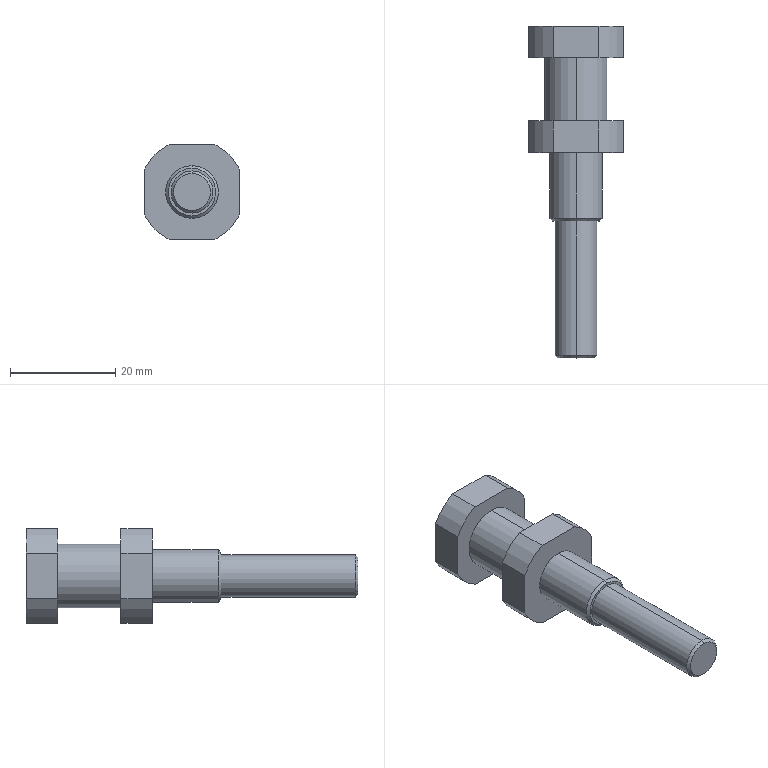Component | SolidWorks | ClampingAssembly-1_A81-1 | 1 solid | 32 faces | box 18 x 63 x 18 mm | volume 7166 mm3 | cylinder 14 | plane 14 | cone 4 | commonest cylinder face diameters 20 x8 8 x2 10 x2 12 x2 | material S45C
build123d program:
from build123d import *

# Parameters (mm, degrees)
SKETCH1_R           = 6
BOSS_EXTRUDE1_DEPTH = 6
SKETCH2_R           = 10
BOSS_EXTRUDE3_DEPTH = 6
SKETCH4_OUTSIDE_W   = 29.418
SKETCH4_OUTSIDE_H   = 29.418
SKETCH4_OUTSIDE_W_2 = 18
SKETCH4_OUTSIDE_H_2 = 18
CUT_EXTRUDE1_DEPTH  = 28.857
SKETCH5_R           = 5
BOSS_EXTRUDE4_DEPTH = 13
CHAMFER1_SIZE       = 0.5
SKETCH6_R           = 4
BOSS_EXTRUDE5_DEPTH = 26
CHAMFER2_SIZE       = 0.5


with BuildPart() as part:
    # Sketch1 → Boss-Extrude1 (new, symmetric)
    with BuildSketch(Plane(origin=(0, 0, 0), x_dir=(0, 0, -1), z_dir=(1, 0, 0))):
        Circle(SKETCH1_R)
    extrude(amount=BOSS_EXTRUDE1_DEPTH, both=True)

    # Sketch2 → Boss-Extrude3 (add)
    with BuildSketch(Plane.ZY.offset(6)):
        Circle(SKETCH2_R)
    boss_extrude3 = extrude(amount=BOSS_EXTRUDE3_DEPTH)

    # Mirror2: Boss-Extrude3 across plane
    add(boss_extrude3.mirror(Plane(origin=(0, 0, 0), x_dir=(0, 0, 1), z_dir=(1, 0, 0))))

    # Sketch4 outside → Cut-Extrude1 (cut, through all)
    with BuildSketch(Plane.ZY.offset(12)):
        Rectangle(SKETCH4_OUTSIDE_W, SKETCH4_OUTSIDE_H)
        Rectangle(SKETCH4_OUTSIDE_W_2, SKETCH4_OUTSIDE_H_2, mode=Mode.SUBTRACT)
    extrude(amount=-CUT_EXTRUDE1_DEPTH, mode=Mode.SUBTRACT)

    # Sketch5 → Boss-Extrude4 (add)
    with BuildSketch(Plane(origin=(12, 0, 0), x_dir=(0, 0, -1), z_dir=(1, 0, 0))):
        with Locations(Location((0, 0, 0), (0, 0, 180))):
            Circle(SKETCH5_R)
    extrude(amount=BOSS_EXTRUDE4_DEPTH)

    # Chamfer1
    chamfer1_edges = [part.edges().sort_by_distance(p)[0] for p in [
        (25, 0, -5),
    ]]
    chamfer(chamfer1_edges, length=CHAMFER1_SIZE)

    # Sketch6 → Boss-Extrude5 (add)
    with BuildSketch(Plane(origin=(25, 0, 0), x_dir=(0, 0, -1), z_dir=(1, 0, 0))):
        with Locations(Location((0, 0, 0), (0, 0, 180))):
            Circle(SKETCH6_R)
    extrude(amount=BOSS_EXTRUDE5_DEPTH)

    # Chamfer2
    chamfer2_edges = [part.edges().sort_by_distance(p)[0] for p in [
        (51, 0, -4),
    ]]
    chamfer(chamfer2_edges, length=CHAMFER2_SIZE)


solid = part.part

# Placed as in the assembly
solid = solid.moved(Location((10.449, 44.036, -37.5), (0, 0, -90)))
STEP:
#1=CARTESIAN_POINT('',(0.4114,-0.2742,-1.614));
#2=VERTEX_POINT('',#1);
#3=CARTESIAN_POINT('',(0.4114,-0.2742,-1.339));
#4=VERTEX_POINT('',#3);
#5=CARTESIAN_POINT('',(0.4114,-0.2742,-1.476));
#6=DIRECTION('',(-0.,-1.,0.));
#7=DIRECTION('',(-0.,-0.,-1.));
#8=AXIS2_PLACEMENT_3D('',#5,#6,#7);
#9=CIRCLE('',#8,0.1378);
#10=EDGE_CURVE('',#2,#4,#9,.T.);
#11=ORIENTED_EDGE('',*,*,#10,.F.);
#12=CARTESIAN_POINT('',(0.4114,-0.2545,-1.634));
#13=VERTEX_POINT('',#12);
#14=CARTESIAN_POINT('',(0.4114,-0.2742,-1.614));
#15=DIRECTION('',(-0.,0.7071,-0.7071));
#16=VECTOR('',#15,39.37);
#17=LINE('',#14,#16);
#18=EDGE_CURVE('',#2,#13,#17,.T.);
#19=ORIENTED_EDGE('',*,*,#18,.T.);
#20=CARTESIAN_POINT('',(0.4114,-0.2545,-1.319));
#21=VERTEX_POINT('',#20);
#22=CARTESIAN_POINT('',(0.4114,-0.2545,-1.476));
#23=DIRECTION('',(0.,1.,-0.));
#24=DIRECTION('',(-0.,-0.,-1.));
#25=AXIS2_PLACEMENT_3D('',#22,#23,#24);
#26=CIRCLE('',#25,0.1575);
#27=EDGE_CURVE('',#21,#13,#26,.T.);
#28=ORIENTED_EDGE('',*,*,#27,.F.);
#29=CARTESIAN_POINT('',(0.4114,-0.2742,-1.339));
#30=DIRECTION('',(0.,0.7071,0.7071));
#31=VECTOR('',#30,39.37);
#32=LINE('',#29,#31);
#33=EDGE_CURVE('',#4,#21,#32,.T.);
#34=ORIENTED_EDGE('',*,*,#33,.F.);
#35=EDGE_LOOP('',(#11,#19,#28,#34));
#36=FACE_OUTER_BOUND('',#35,.T.);
#37=CARTESIAN_POINT('',(0.4114,-0.2742,-1.476));
#38=DIRECTION('',(0.,1.,-0.));
#39=DIRECTION('',(0.,0.,1.));
#40=AXIS2_PLACEMENT_3D('',#37,#38,#39);
#41=CONICAL_SURFACE('',#40,0.1378,0.7854);
#42=ADVANCED_FACE('',(#36),#41,.T.);
#43=ORIENTED_EDGE('',*,*,#27,.T.);
#44=CARTESIAN_POINT('',(0.4114,0.7494,-1.634));
#45=VERTEX_POINT('',#44);
#46=CARTESIAN_POINT('',(0.4114,-0.2742,-1.634));
#47=DIRECTION('',(0.,1.,-0.));
#48=VECTOR('',#47,39.37);
#49=LINE('',#46,#48);
#50=EDGE_CURVE('',#13,#45,#49,.T.);
#51=ORIENTED_EDGE('',*,*,#50,.T.);
#52=CARTESIAN_POINT('',(0.4114,0.7494,-1.319));
#53=VERTEX_POINT('',#52);
#54=CARTESIAN_POINT('',(0.4114,0.7494,-1.476));
#55=DIRECTION('',(-0.,-1.,0.));
#56=DIRECTION('',(-0.,0.,-1.));
#57=AXIS2_PLACEMENT_3D('',#54,#55,#56);
#58=CIRCLE('',#57,0.1575);
#59=EDGE_CURVE('',#45,#53,#58,.T.);
#60=ORIENTED_EDGE('',*,*,#59,.T.);
#61=CARTESIAN_POINT('',(0.4114,-0.2742,-1.319));
#62=DIRECTION('',(0.,1.,-0.));
#63=VECTOR('',#62,39.37);
#64=LINE('',#61,#63);
#65=EDGE_CURVE('',#21,#53,#64,.T.);
#66=ORIENTED_EDGE('',*,*,#65,.F.);
#67=EDGE_LOOP('',(#43,#51,#60,#66));
#68=FACE_OUTER_BOUND('',#67,.T.);
#69=CARTESIAN_POINT('',(0.4114,-0.2742,-1.476));
#70=DIRECTION('',(0.,1.,-0.));
#71=DIRECTION('',(0.,0.,1.));
#72=AXIS2_PLACEMENT_3D('',#69,#70,#71);
#73=CYLINDRICAL_SURFACE('',#72,0.1575);
#74=ADVANCED_FACE('',(#68),#73,.T.);
#75=CARTESIAN_POINT('',(0.4114,0.7494,-1.654));
#76=VERTEX_POINT('',#75);
#77=CARTESIAN_POINT('',(0.4114,0.7494,-1.299));
#78=VERTEX_POINT('',#77);
#79=CARTESIAN_POINT('',(0.4114,0.7494,-1.476));
#80=DIRECTION('',(-0.,-1.,0.));
#81=DIRECTION('',(-0.,0.,-1.));
#82=AXIS2_PLACEMENT_3D('',#79,#80,#81);
#83=CIRCLE('',#82,0.1772);
#84=EDGE_CURVE('',#76,#78,#83,.T.);
#85=ORIENTED_EDGE('',*,*,#84,.F.);
#86=CARTESIAN_POINT('',(0.4114,0.7691,-1.673));
#87=VERTEX_POINT('',#86);
#88=CARTESIAN_POINT('',(0.4114,0.7494,-1.654));
#89=DIRECTION('',(-0.,0.7071,-0.7071));
#90=VECTOR('',#89,39.37);
#91=LINE('',#88,#90);
#92=EDGE_CURVE('',#76,#87,#91,.T.);
#93=ORIENTED_EDGE('',*,*,#92,.T.);
#94=CARTESIAN_POINT('',(0.4114,0.7691,-1.28));
#95=VERTEX_POINT('',#94);
#96=CARTESIAN_POINT('',(0.4114,0.7691,-1.476));
#97=DIRECTION('',(0.,1.,-0.));
#98=DIRECTION('',(-0.,0.,-1.));
#99=AXIS2_PLACEMENT_3D('',#96,#97,#98);
#100=CIRCLE('',#99,0.1969);
#101=EDGE_CURVE('',#95,#87,#100,.T.);
#102=ORIENTED_EDGE('',*,*,#101,.F.);
#103=CARTESIAN_POINT('',(0.4114,0.7494,-1.299));
#104=DIRECTION('',(0.,0.7071,0.7071));
#105=VECTOR('',#104,39.37);
#106=LINE('',#103,#105);
#107=EDGE_CURVE('',#78,#95,#106,.T.);
#108=ORIENTED_EDGE('',*,*,#107,.F.);
#109=EDGE_LOOP('',(#85,#93,#102,#108));
#110=FACE_OUTER_BOUND('',#109,.T.);
#111=CARTESIAN_POINT('',(0.4114,0.7494,-1.476));
#112=DIRECTION('',(0.,1.,-0.));
#113=DIRECTION('',(0.,0.,1.));
#114=AXIS2_PLACEMENT_3D('',#111,#112,#113);
#115=CONICAL_SURFACE('',#114,0.1772,0.7854);
#116=ADVANCED_FACE('',(#110),#115,.T.);
#117=ORIENTED_EDGE('',*,*,#101,.T.);
#118=CARTESIAN_POINT('',(0.4114,1.261,-1.673));
#119=VERTEX_POINT('',#118);
#120=CARTESIAN_POINT('',(0.4114,0.7494,-1.673));
#121=DIRECTION('',(0.,1.,-0.));
#122=VECTOR('',#121,39.37);
#123=LINE('',#120,#122);
#124=EDGE_CURVE('',#87,#119,#123,.T.);
#125=ORIENTED_EDGE('',*,*,#124,.T.);
#126=CARTESIAN_POINT('',(0.4114,1.261,-1.28));
#127=VERTEX_POINT('',#126);
#128=CARTESIAN_POINT('',(0.4114,1.261,-1.476));
#129=DIRECTION('',(-0.,-1.,0.));
#130=DIRECTION('',(-0.,0.,-1.));
#131=AXIS2_PLACEMENT_3D('',#128,#129,#130);
#132=CIRCLE('',#131,0.1969);
#133=EDGE_CURVE('',#119,#127,#132,.T.);
#134=ORIENTED_EDGE('',*,*,#133,.T.);
#135=CARTESIAN_POINT('',(0.4114,0.7494,-1.28));
#136=DIRECTION('',(0.,1.,-0.));
#137=VECTOR('',#136,39.37);
#138=LINE('',#135,#137);
#139=EDGE_CURVE('',#95,#127,#138,.T.);
#140=ORIENTED_EDGE('',*,*,#139,.F.);
#141=EDGE_LOOP('',(#117,#125,#134,#140));
#142=FACE_OUTER_BOUND('',#141,.T.);
#143=CARTESIAN_POINT('',(0.4114,0.7494,-1.476));
#144=DIRECTION('',(0.,1.,-0.));
#145=DIRECTION('',(0.,0.,1.));
#146=AXIS2_PLACEMENT_3D('',#143,#144,#145);
#147=CYLINDRICAL_SURFACE('',#146,0.1969);
#148=ADVANCED_FACE('',(#142),#147,.T.);
#149=CARTESIAN_POINT('',(0.4114,1.497,-1.713));
#150=VERTEX_POINT('',#149);
#151=CARTESIAN_POINT('',(0.4114,1.497,-1.24));
#152=VERTEX_POINT('',#151);
#153=CARTESIAN_POINT('',(0.4114,1.497,-1.476));
#154=DIRECTION('',(-0.,-1.,0.));
#155=DIRECTION('',(-0.,0.,-1.));
#156=AXIS2_PLACEMENT_3D('',#153,#154,#155);
#157=CIRCLE('',#156,0.2362);
#158=EDGE_CURVE('',#150,#152,#157,.T.);
#159=ORIENTED_EDGE('',*,*,#158,.F.);
#160=CARTESIAN_POINT('',(0.4114,1.97,-1.713));
#161=VERTEX_POINT('',#160);
#162=CARTESIAN_POINT('',(0.4114,1.497,-1.713));
#163=DIRECTION('',(0.,1.,-0.));
#164=VECTOR('',#163,39.37);
#165=LINE('',#162,#164);
#166=EDGE_CURVE('',#150,#161,#165,.T.);
#167=ORIENTED_EDGE('',*,*,#166,.T.);
#168=CARTESIAN_POINT('',(0.4114,1.97,-1.24));
#169=VERTEX_POINT('',#168);
#170=CARTESIAN_POINT('',(0.4114,1.97,-1.476));
#171=DIRECTION('',(-0.,-1.,0.));
#172=DIRECTION('',(-0.,0.,-1.));
#173=AXIS2_PLACEMENT_3D('',#170,#171,#172);
#174=CIRCLE('',#173,0.2362);
#175=EDGE_CURVE('',#161,#169,#174,.T.);
#176=ORIENTED_EDGE('',*,*,#175,.T.);
#177=CARTESIAN_POINT('',(0.4114,1.497,-1.24));
#178=DIRECTION('',(0.,1.,-0.));
#179=VECTOR('',#178,39.37);
#180=LINE('',#177,#179);
#181=EDGE_CURVE('',#152,#169,#180,.T.);
#182=ORIENTED_EDGE('',*,*,#181,.F.);
#183=EDGE_LOOP('',(#159,#167,#176,#182));
#184=FACE_OUTER_BOUND('',#183,.T.);
#185=CARTESIAN_POINT('',(0.4114,1.497,-1.476));
#186=DIRECTION('',(0.,1.,-0.));
#187=DIRECTION('',(0.,0.,1.));
#188=AXIS2_PLACEMENT_3D('',#185,#186,#187);
#189=CYLINDRICAL_SURFACE('',#188,0.2362);
#190=ADVANCED_FACE('',(#184),#189,.T.);
#191=CARTESIAN_POINT('',(0.2398,2.206,-1.122));
#192=VERTEX_POINT('',#191);
#193=CARTESIAN_POINT('',(0.2398,1.97,-1.122));
#194=VERTEX_POINT('',#193);
#195=CARTESIAN_POINT('',(0.2398,2.206,-1.122));
#196=DIRECTION('',(-0.,-1.,0.));
#197=VECTOR('',#196,39.37);
#198=LINE('',#195,#197);
#199=EDGE_CURVE('',#192,#194,#198,.T.);
#200=ORIENTED_EDGE('',*,*,#199,.F.);
#201=CARTESIAN_POINT('',(0.05706,2.206,-1.305));
#202=VERTEX_POINT('',#201);
#203=CARTESIAN_POINT('',(0.4114,2.206,-1.476));
#204=DIRECTION('',(0.,1.,-0.));
#205=DIRECTION('',(0.,0.,1.));
#206=AXIS2_PLACEMENT_3D('',#203,#204,#205);
#207=CIRCLE('',#206,0.3937);
#208=EDGE_CURVE('',#202,#192,#207,.T.);
#209=ORIENTED_EDGE('',*,*,#208,.F.);
#210=CARTESIAN_POINT('',(0.05706,1.97,-1.305));
#211=VERTEX_POINT('',#210);
#212=CARTESIAN_POINT('',(0.05706,2.206,-1.305));
#213=DIRECTION('',(0.,1.,-0.));
#214=VECTOR('',#213,39.37);
#215=LINE('',#212,#214);
#216=EDGE_CURVE('',#211,#202,#215,.T.);
#217=ORIENTED_EDGE('',*,*,#216,.F.);
#218=CARTESIAN_POINT('',(0.4114,1.97,-1.476));
#219=DIRECTION('',(0.,1.,-0.));
#220=DIRECTION('',(0.,0.,1.));
#221=AXIS2_PLACEMENT_3D('',#218,#219,#220);
#222=CIRCLE('',#221,0.3937);
#223=EDGE_CURVE('',#211,#194,#222,.T.);
#224=ORIENTED_EDGE('',*,*,#223,.T.);
#225=EDGE_LOOP('',(#200,#209,#217,#224));
#226=FACE_OUTER_BOUND('',#225,.T.);
#227=CARTESIAN_POINT('',(0.4114,2.206,-1.476));
#228=DIRECTION('',(-0.,-1.,0.));
#229=DIRECTION('',(-0.,0.,-1.));
#230=AXIS2_PLACEMENT_3D('',#227,#228,#229);
#231=CYLINDRICAL_SURFACE('',#230,0.3937);
#232=ADVANCED_FACE('',(#226),#231,.T.);
#233=CARTESIAN_POINT('',(0.583,1.97,-1.122));
#234=VERTEX_POINT('',#233);
#235=CARTESIAN_POINT('',(0.583,2.206,-1.122));
#236=VERTEX_POINT('',#235);
#237=CARTESIAN_POINT('',(0.583,2.206,-1.122));
#238=DIRECTION('',(0.,1.,-0.));
#239=VECTOR('',#238,39.37);
#240=LINE('',#237,#239);
#241=EDGE_CURVE('',#234,#236,#240,.T.);
#242=ORIENTED_EDGE('',*,*,#241,.F.);
#243=CARTESIAN_POINT('',(0.7657,1.97,-1.305));
#244=VERTEX_POINT('',#243);
#245=CARTESIAN_POINT('',(0.4114,1.97,-1.476));
#246=DIRECTION('',(0.,1.,-0.));
#247=DIRECTION('',(0.,0.,1.));
#248=AXIS2_PLACEMENT_3D('',#245,#246,#247);
#249=CIRCLE('',#248,0.3937);
#250=EDGE_CURVE('',#234,#244,#249,.T.);
#251=ORIENTED_EDGE('',*,*,#250,.T.);
#252=CARTESIAN_POINT('',(0.7657,2.206,-1.305));
#253=VERTEX_POINT('',#252);
#254=CARTESIAN_POINT('',(0.7657,2.206,-1.305));
#255=DIRECTION('',(-0.,-1.,0.));
#256=VECTOR('',#255,39.37);
#257=LINE('',#254,#256);
#258=EDGE_CURVE('',#253,#244,#257,.T.);
#259=ORIENTED_EDGE('',*,*,#258,.F.);
#260=CARTESIAN_POINT('',(0.4114,2.206,-1.476));
#261=DIRECTION('',(0.,1.,-0.));
#262=DIRECTION('',(0.,0.,1.));
#263=AXIS2_PLACEMENT_3D('',#260,#261,#262);
#264=CIRCLE('',#263,0.3937);
#265=EDGE_CURVE('',#236,#253,#264,.T.);
#266=ORIENTED_EDGE('',*,*,#265,.F.);
#267=EDGE_LOOP('',(#242,#251,#259,#266));
#268=FACE_OUTER_BOUND('',#267,.T.);
#269=CARTESIAN_POINT('',(0.4114,2.206,-1.476));
#270=DIRECTION('',(-0.,-1.,0.));
#271=DIRECTION('',(-0.,0.,-1.));
#272=AXIS2_PLACEMENT_3D('',#269,#270,#271);
#273=CYLINDRICAL_SURFACE('',#272,0.3937);
#274=ADVANCED_FACE('',(#268),#273,.T.);
#275=CARTESIAN_POINT('',(0.05706,2.206,-1.648));
#276=VERTEX_POINT('',#275);
#277=CARTESIAN_POINT('',(0.05706,1.97,-1.648));
#278=VERTEX_POINT('',#277);
#279=CARTESIAN_POINT('',(0.05706,2.206,-1.648));
#280=DIRECTION('',(-0.,-1.,0.));
#281=VECTOR('',#280,39.37);
#282=LINE('',#279,#281);
#283=EDGE_CURVE('',#276,#278,#282,.T.);
#284=ORIENTED_EDGE('',*,*,#283,.F.);
#285=CARTESIAN_POINT('',(0.2398,2.206,-1.831));
#286=VERTEX_POINT('',#285);
#287=CARTESIAN_POINT('',(0.4114,2.206,-1.476));
#288=DIRECTION('',(0.,1.,-0.));
#289=DIRECTION('',(0.,0.,1.));
#290=AXIS2_PLACEMENT_3D('',#287,#288,#289);
#291=CIRCLE('',#290,0.3937);
#292=EDGE_CURVE('',#286,#276,#291,.T.);
#293=ORIENTED_EDGE('',*,*,#292,.F.);
#294=CARTESIAN_POINT('',(0.2398,1.97,-1.831));
#295=VERTEX_POINT('',#294);
#296=CARTESIAN_POINT('',(0.2398,2.206,-1.831));
#297=DIRECTION('',(0.,1.,-0.));
#298=VECTOR('',#297,39.37);
#299=LINE('',#296,#298);
#300=EDGE_CURVE('',#295,#286,#299,.T.);
#301=ORIENTED_EDGE('',*,*,#300,.F.);
#302=CARTESIAN_POINT('',(0.4114,1.97,-1.476));
#303=DIRECTION('',(0.,1.,-0.));
#304=DIRECTION('',(0.,0.,1.));
#305=AXIS2_PLACEMENT_3D('',#302,#303,#304);
#306=CIRCLE('',#305,0.3937);
#307=EDGE_CURVE('',#295,#278,#306,.T.);
#308=ORIENTED_EDGE('',*,*,#307,.T.);
#309=EDGE_LOOP('',(#284,#293,#301,#308));
#310=FACE_OUTER_BOUND('',#309,.T.);
#311=CARTESIAN_POINT('',(0.4114,2.206,-1.476));
#312=DIRECTION('',(-0.,-1.,0.));
#313=DIRECTION('',(-0.,0.,-1.));
#314=AXIS2_PLACEMENT_3D('',#311,#312,#313);
#315=CYLINDRICAL_SURFACE('',#314,0.3937);
#316=ADVANCED_FACE('',(#310),#315,.T.);
#317=CARTESIAN_POINT('',(0.583,2.206,-1.831));
#318=VERTEX_POINT('',#317);
#319=CARTESIAN_POINT('',(0.583,1.97,-1.831));
#320=VERTEX_POINT('',#319);
#321=CARTESIAN_POINT('',(0.583,2.206,-1.831));
#322=DIRECTION('',(-0.,-1.,0.));
#323=VECTOR('',#322,39.37);
#324=LINE('',#321,#323);
#325=EDGE_CURVE('',#318,#320,#324,.T.);
#326=ORIENTED_EDGE('',*,*,#325,.F.);
#327=CARTESIAN_POINT('',(0.7657,2.206,-1.648));
#328=VERTEX_POINT('',#327);
#329=CARTESIAN_POINT('',(0.4114,2.206,-1.476));
#330=DIRECTION('',(0.,1.,-0.));
#331=DIRECTION('',(0.,0.,1.));
#332=AXIS2_PLACEMENT_3D('',#329,#330,#331);
#333=CIRCLE('',#332,0.3937);
#334=EDGE_CURVE('',#328,#318,#333,.T.);
#335=ORIENTED_EDGE('',*,*,#334,.F.);
#336=CARTESIAN_POINT('',(0.7657,1.97,-1.648));
#337=VERTEX_POINT('',#336);
#338=CARTESIAN_POINT('',(0.7657,2.206,-1.648));
#339=DIRECTION('',(0.,1.,-0.));
#340=VECTOR('',#339,39.37);
#341=LINE('',#338,#340);
#342=EDGE_CURVE('',#337,#328,#341,.T.);
#343=ORIENTED_EDGE('',*,*,#342,.F.);
#344=CARTESIAN_POINT('',(0.4114,1.97,-1.476));
#345=DIRECTION('',(0.,1.,-0.));
#346=DIRECTION('',(0.,0.,1.));
#347=AXIS2_PLACEMENT_3D('',#344,#345,#346);
#348=CIRCLE('',#347,0.3937);
#349=EDGE_CURVE('',#337,#320,#348,.T.);
#350=ORIENTED_EDGE('',*,*,#349,.T.);
#351=EDGE_LOOP('',(#326,#335,#343,#350));
#352=FACE_OUTER_BOUND('',#351,.T.);
#353=CARTESIAN_POINT('',(0.4114,2.206,-1.476));
#354=DIRECTION('',(-0.,-1.,0.));
#355=DIRECTION('',(-0.,0.,-1.));
#356=AXIS2_PLACEMENT_3D('',#353,#354,#355);
#357=CYLINDRICAL_SURFACE('',#356,0.3937);
#358=ADVANCED_FACE('',(#352),#357,.T.);
#359=ORIENTED_EDGE('',*,*,#208,.T.);
#360=CARTESIAN_POINT('',(0.7657,2.206,-1.122));
#361=DIRECTION('',(1.,-0.,-0.));
#362=VECTOR('',#361,39.37);
#363=LINE('',#360,#362);
#364=EDGE_CURVE('',#192,#236,#363,.T.);
#365=ORIENTED_EDGE('',*,*,#364,.T.);
#366=ORIENTED_EDGE('',*,*,#265,.T.);
#367=CARTESIAN_POINT('',(0.7657,2.206,-1.831));
#368=DIRECTION('',(-0.,-0.,-1.));
#369=VECTOR('',#368,39.37);
#370=LINE('',#367,#369);
#371=EDGE_CURVE('',#253,#328,#370,.T.);
#372=ORIENTED_EDGE('',*,*,#371,.T.);
#373=ORIENTED_EDGE('',*,*,#334,.T.);
#374=CARTESIAN_POINT('',(0.7657,2.206,-1.831));
#375=DIRECTION('',(-1.,0.,0.));
#376=VECTOR('',#375,39.37);
#377=LINE('',#374,#376);
#378=EDGE_CURVE('',#318,#286,#377,.T.);
#379=ORIENTED_EDGE('',*,*,#378,.T.);
#380=ORIENTED_EDGE('',*,*,#292,.T.);
#381=CARTESIAN_POINT('',(0.05706,2.206,-1.831));
#382=DIRECTION('',(0.,0.,1.));
#383=VECTOR('',#382,39.37);
#384=LINE('',#381,#383);
#385=EDGE_CURVE('',#276,#202,#384,.T.);
#386=ORIENTED_EDGE('',*,*,#385,.T.);
#387=EDGE_LOOP('',(#359,#365,#366,#372,#373,#379,#380,#386));
#388=FACE_OUTER_BOUND('',#387,.T.);
#389=CARTESIAN_POINT('',(0.4114,2.206,-1.476));
#390=DIRECTION('',(0.,1.,-0.));
#391=DIRECTION('',(0.,0.,1.));
#392=AXIS2_PLACEMENT_3D('',#389,#390,#391);
#393=PLANE('',#392);
#394=ADVANCED_FACE('',(#388),#393,.T.);
#395=CARTESIAN_POINT('',(0.4114,1.97,-1.476));
#396=DIRECTION('',(-0.,-1.,0.));
#397=DIRECTION('',(-0.,0.,-1.));
#398=AXIS2_PLACEMENT_3D('',#395,#396,#397);
#399=CIRCLE('',#398,0.2362);
#400=EDGE_CURVE('',#169,#161,#399,.T.);
#401=ORIENTED_EDGE('',*,*,#400,.F.);
#402=ORIENTED_EDGE('',*,*,#175,.F.);
#403=EDGE_LOOP('',(#401,#402));
#404=FACE_BOUND('',#403,.T.);
#405=CARTESIAN_POINT('',(0.4114,1.97,-1.122));
#406=DIRECTION('',(1.,-0.,-0.));
#407=VECTOR('',#406,39.37);
#408=LINE('',#405,#407);
#409=EDGE_CURVE('',#194,#234,#408,.T.);
#410=ORIENTED_EDGE('',*,*,#409,.F.);
#411=ORIENTED_EDGE('',*,*,#223,.F.);
#412=CARTESIAN_POINT('',(0.05706,1.97,-1.476));
#413=DIRECTION('',(0.,0.,1.));
#414=VECTOR('',#413,39.37);
#415=LINE('',#412,#414);
#416=EDGE_CURVE('',#278,#211,#415,.T.);
#417=ORIENTED_EDGE('',*,*,#416,.F.);
#418=ORIENTED_EDGE('',*,*,#307,.F.);
#419=CARTESIAN_POINT('',(0.4114,1.97,-1.831));
#420=DIRECTION('',(-1.,0.,0.));
#421=VECTOR('',#420,39.37);
#422=LINE('',#419,#421);
#423=EDGE_CURVE('',#320,#295,#422,.T.);
#424=ORIENTED_EDGE('',*,*,#423,.F.);
#425=ORIENTED_EDGE('',*,*,#349,.F.);
#426=CARTESIAN_POINT('',(0.7657,1.97,-1.476));
#427=DIRECTION('',(-0.,-0.,-1.));
#428=VECTOR('',#427,39.37);
#429=LINE('',#426,#428);
#430=EDGE_CURVE('',#244,#337,#429,.T.);
#431=ORIENTED_EDGE('',*,*,#430,.F.);
#432=ORIENTED_EDGE('',*,*,#250,.F.);
#433=EDGE_LOOP('',(#410,#411,#417,#418,#424,#425,#431,#432));
#434=FACE_OUTER_BOUND('',#433,.T.);
#435=CARTESIAN_POINT('',(0.4114,1.97,-1.476));
#436=DIRECTION('',(0.,1.,-0.));
#437=DIRECTION('',(0.,0.,1.));
#438=AXIS2_PLACEMENT_3D('',#435,#436,#437);
#439=PLANE('',#438);
#440=ADVANCED_FACE('',(#404,#434),#439,.F.);
#441=CARTESIAN_POINT('',(0.583,1.497,-1.122));
#442=VERTEX_POINT('',#441);
#443=CARTESIAN_POINT('',(0.7657,1.497,-1.305));
#444=VERTEX_POINT('',#443);
#445=CARTESIAN_POINT('',(0.4114,1.497,-1.476));
#446=DIRECTION('',(0.,1.,-0.));
#447=DIRECTION('',(0.,0.,1.));
#448=AXIS2_PLACEMENT_3D('',#445,#446,#447);
#449=CIRCLE('',#448,0.3937);
#450=EDGE_CURVE('',#442,#444,#449,.T.);
#451=ORIENTED_EDGE('',*,*,#450,.F.);
#452=CARTESIAN_POINT('',(0.583,1.261,-1.122));
#453=VERTEX_POINT('',#452);
#454=CARTESIAN_POINT('',(0.583,1.261,-1.122));
#455=DIRECTION('',(-0.,-1.,0.));
#456=VECTOR('',#455,39.37);
#457=LINE('',#454,#456);
#458=EDGE_CURVE('',#442,#453,#457,.T.);
#459=ORIENTED_EDGE('',*,*,#458,.T.);
#460=CARTESIAN_POINT('',(0.7657,1.261,-1.305));
#461=VERTEX_POINT('',#460);
#462=CARTESIAN_POINT('',(0.4114,1.261,-1.476));
#463=DIRECTION('',(0.,1.,-0.));
#464=DIRECTION('',(0.,0.,1.));
#465=AXIS2_PLACEMENT_3D('',#462,#463,#464);
#466=CIRCLE('',#465,0.3937);
#467=EDGE_CURVE('',#453,#461,#466,.T.);
#468=ORIENTED_EDGE('',*,*,#467,.T.);
#469=CARTESIAN_POINT('',(0.7657,1.261,-1.305));
#470=DIRECTION('',(0.,1.,-0.));
#471=VECTOR('',#470,39.37);
#472=LINE('',#469,#471);
#473=EDGE_CURVE('',#461,#444,#472,.T.);
#474=ORIENTED_EDGE('',*,*,#473,.T.);
#475=EDGE_LOOP('',(#451,#459,#468,#474));
#476=FACE_OUTER_BOUND('',#475,.T.);
#477=CARTESIAN_POINT('',(0.4114,1.261,-1.476));
#478=DIRECTION('',(0.,1.,-0.));
#479=DIRECTION('',(0.,0.,1.));
#480=AXIS2_PLACEMENT_3D('',#477,#478,#479);
#481=CYLINDRICAL_SURFACE('',#480,0.3937);
#482=ADVANCED_FACE('',(#476),#481,.T.);
#483=CARTESIAN_POINT('',(0.05706,1.261,-1.305));
#484=VERTEX_POINT('',#483);
#485=CARTESIAN_POINT('',(0.2398,1.261,-1.122));
#486=VERTEX_POINT('',#485);
#487=CARTESIAN_POINT('',(0.4114,1.261,-1.476));
#488=DIRECTION('',(0.,1.,-0.));
#489=DIRECTION('',(0.,0.,1.));
#490=AXIS2_PLACEMENT_3D('',#487,#488,#489);
#491=CIRCLE('',#490,0.3937);
#492=EDGE_CURVE('',#484,#486,#491,.T.);
#493=ORIENTED_EDGE('',*,*,#492,.T.);
#494=CARTESIAN_POINT('',(0.2398,1.497,-1.122));
#495=VERTEX_POINT('',#494);
#496=CARTESIAN_POINT('',(0.2398,1.261,-1.122));
#497=DIRECTION('',(0.,1.,-0.));
#498=VECTOR('',#497,39.37);
#499=LINE('',#496,#498);
#500=EDGE_CURVE('',#486,#495,#499,.T.);
#501=ORIENTED_EDGE('',*,*,#500,.T.);
#502=CARTESIAN_POINT('',(0.05706,1.497,-1.305));
#503=VERTEX_POINT('',#502);
#504=CARTESIAN_POINT('',(0.4114,1.497,-1.476));
#505=DIRECTION('',(0.,1.,-0.));
#506=DIRECTION('',(0.,0.,1.));
#507=AXIS2_PLACEMENT_3D('',#504,#505,#506);
#508=CIRCLE('',#507,0.3937);
#509=EDGE_CURVE('',#503,#495,#508,.T.);
#510=ORIENTED_EDGE('',*,*,#509,.F.);
#511=CARTESIAN_POINT('',(0.05706,1.261,-1.305));
#512=DIRECTION('',(-0.,-1.,0.));
#513=VECTOR('',#512,39.37);
#514=LINE('',#511,#513);
#515=EDGE_CURVE('',#503,#484,#514,.T.);
#516=ORIENTED_EDGE('',*,*,#515,.T.);
#517=EDGE_LOOP('',(#493,#501,#510,#516));
#518=FACE_OUTER_BOUND('',#517,.T.);
#519=CARTESIAN_POINT('',(0.4114,1.261,-1.476));
#520=DIRECTION('',(0.,1.,-0.));
#521=DIRECTION('',(0.,0.,1.));
#522=AXIS2_PLACEMENT_3D('',#519,#520,#521);
#523=CYLINDRICAL_SURFACE('',#522,0.3937);
#524=ADVANCED_FACE('',(#518),#523,.T.);
#525=CARTESIAN_POINT('',(0.2398,1.261,-1.831));
#526=VERTEX_POINT('',#525);
#527=CARTESIAN_POINT('',(0.05706,1.261,-1.648));
#528=VERTEX_POINT('',#527);
#529=CARTESIAN_POINT('',(0.4114,1.261,-1.476));
#530=DIRECTION('',(0.,1.,-0.));
#531=DIRECTION('',(0.,0.,1.));
#532=AXIS2_PLACEMENT_3D('',#529,#530,#531);
#533=CIRCLE('',#532,0.3937);
#534=EDGE_CURVE('',#526,#528,#533,.T.);
#535=ORIENTED_EDGE('',*,*,#534,.T.);
#536=CARTESIAN_POINT('',(0.05706,1.497,-1.648));
#537=VERTEX_POINT('',#536);
#538=CARTESIAN_POINT('',(0.05706,1.261,-1.648));
#539=DIRECTION('',(0.,1.,-0.));
#540=VECTOR('',#539,39.37);
#541=LINE('',#538,#540);
#542=EDGE_CURVE('',#528,#537,#541,.T.);
#543=ORIENTED_EDGE('',*,*,#542,.T.);
#544=CARTESIAN_POINT('',(0.2398,1.497,-1.831));
#545=VERTEX_POINT('',#544);
#546=CARTESIAN_POINT('',(0.4114,1.497,-1.476));
#547=DIRECTION('',(0.,1.,-0.));
#548=DIRECTION('',(0.,0.,1.));
#549=AXIS2_PLACEMENT_3D('',#546,#547,#548);
#550=CIRCLE('',#549,0.3937);
#551=EDGE_CURVE('',#545,#537,#550,.T.);
#552=ORIENTED_EDGE('',*,*,#551,.F.);
#553=CARTESIAN_POINT('',(0.2398,1.261,-1.831));
#554=DIRECTION('',(-0.,-1.,0.));
#555=VECTOR('',#554,39.37);
#556=LINE('',#553,#555);
#557=EDGE_CURVE('',#545,#526,#556,.T.);
#558=ORIENTED_EDGE('',*,*,#557,.T.);
#559=EDGE_LOOP('',(#535,#543,#552,#558));
#560=FACE_OUTER_BOUND('',#559,.T.);
#561=CARTESIAN_POINT('',(0.4114,1.261,-1.476));
#562=DIRECTION('',(0.,1.,-0.));
#563=DIRECTION('',(0.,0.,1.));
#564=AXIS2_PLACEMENT_3D('',#561,#562,#563);
#565=CYLINDRICAL_SURFACE('',#564,0.3937);
#566=ADVANCED_FACE('',(#560),#565,.T.);
#567=CARTESIAN_POINT('',(0.7657,1.261,-1.648));
#568=VERTEX_POINT('',#567);
#569=CARTESIAN_POINT('',(0.583,1.261,-1.831));
#570=VERTEX_POINT('',#569);
#571=CARTESIAN_POINT('',(0.4114,1.261,-1.476));
#572=DIRECTION('',(0.,1.,-0.));
#573=DIRECTION('',(0.,0.,1.));
#574=AXIS2_PLACEMENT_3D('',#571,#572,#573);
#575=CIRCLE('',#574,0.3937);
#576=EDGE_CURVE('',#568,#570,#575,.T.);
#577=ORIENTED_EDGE('',*,*,#576,.T.);
#578=CARTESIAN_POINT('',(0.583,1.497,-1.831));
#579=VERTEX_POINT('',#578);
#580=CARTESIAN_POINT('',(0.583,1.261,-1.831));
#581=DIRECTION('',(0.,1.,-0.));
#582=VECTOR('',#581,39.37);
#583=LINE('',#580,#582);
#584=EDGE_CURVE('',#570,#579,#583,.T.);
#585=ORIENTED_EDGE('',*,*,#584,.T.);
#586=CARTESIAN_POINT('',(0.7657,1.497,-1.648));
#587=VERTEX_POINT('',#586);
#588=CARTESIAN_POINT('',(0.4114,1.497,-1.476));
#589=DIRECTION('',(0.,1.,-0.));
#590=DIRECTION('',(0.,0.,1.));
#591=AXIS2_PLACEMENT_3D('',#588,#589,#590);
#592=CIRCLE('',#591,0.3937);
#593=EDGE_CURVE('',#587,#579,#592,.T.);
#594=ORIENTED_EDGE('',*,*,#593,.F.);
#595=CARTESIAN_POINT('',(0.7657,1.261,-1.648));
#596=DIRECTION('',(-0.,-1.,0.));
#597=VECTOR('',#596,39.37);
#598=LINE('',#595,#597);
#599=EDGE_CURVE('',#587,#568,#598,.T.);
#600=ORIENTED_EDGE('',*,*,#599,.T.);
#601=EDGE_LOOP('',(#577,#585,#594,#600));
#602=FACE_OUTER_BOUND('',#601,.T.);
#603=CARTESIAN_POINT('',(0.4114,1.261,-1.476));
#604=DIRECTION('',(0.,1.,-0.));
#605=DIRECTION('',(0.,0.,1.));
#606=AXIS2_PLACEMENT_3D('',#603,#604,#605);
#607=CYLINDRICAL_SURFACE('',#606,0.3937);
#608=ADVANCED_FACE('',(#602),#607,.T.);
#609=CARTESIAN_POINT('',(0.4114,1.261,-1.476));
#610=DIRECTION('',(-0.,-1.,0.));
#611=DIRECTION('',(-0.,0.,-1.));
#612=AXIS2_PLACEMENT_3D('',#609,#610,#611);
#613=CIRCLE('',#612,0.1969);
#614=EDGE_CURVE('',#127,#119,#613,.T.);
#615=ORIENTED_EDGE('',*,*,#614,.F.);
#616=ORIENTED_EDGE('',*,*,#133,.F.);
#617=EDGE_LOOP('',(#615,#616));
#618=FACE_BOUND('',#617,.T.);
#619=ORIENTED_EDGE('',*,*,#467,.F.);
#620=CARTESIAN_POINT('',(0.7657,1.261,-1.122));
#621=DIRECTION('',(1.,-0.,-0.));
#622=VECTOR('',#621,39.37);
#623=LINE('',#620,#622);
#624=EDGE_CURVE('',#486,#453,#623,.T.);
#625=ORIENTED_EDGE('',*,*,#624,.F.);
#626=ORIENTED_EDGE('',*,*,#492,.F.);
#627=CARTESIAN_POINT('',(0.05706,1.261,-1.831));
#628=DIRECTION('',(0.,0.,1.));
#629=VECTOR('',#628,39.37);
#630=LINE('',#627,#629);
#631=EDGE_CURVE('',#528,#484,#630,.T.);
#632=ORIENTED_EDGE('',*,*,#631,.F.);
#633=ORIENTED_EDGE('',*,*,#534,.F.);
#634=CARTESIAN_POINT('',(0.7657,1.261,-1.831));
#635=DIRECTION('',(-1.,0.,0.));
#636=VECTOR('',#635,39.37);
#637=LINE('',#634,#636);
#638=EDGE_CURVE('',#570,#526,#637,.T.);
#639=ORIENTED_EDGE('',*,*,#638,.F.);
#640=ORIENTED_EDGE('',*,*,#576,.F.);
#641=CARTESIAN_POINT('',(0.7657,1.261,-1.831));
#642=DIRECTION('',(-0.,-0.,-1.));
#643=VECTOR('',#642,39.37);
#644=LINE('',#641,#643);
#645=EDGE_CURVE('',#461,#568,#644,.T.);
#646=ORIENTED_EDGE('',*,*,#645,.F.);
#647=EDGE_LOOP('',(#619,#625,#626,#632,#633,#639,#640,#646));
#648=FACE_OUTER_BOUND('',#647,.T.);
#649=CARTESIAN_POINT('',(0.4114,1.261,-1.476));
#650=DIRECTION('',(-0.,-1.,0.));
#651=DIRECTION('',(0.,0.,1.));
#652=AXIS2_PLACEMENT_3D('',#649,#650,#651);
#653=PLANE('',#652);
#654=ADVANCED_FACE('',(#618,#648),#653,.T.);
#655=CARTESIAN_POINT('',(0.4114,1.497,-1.476));
#656=DIRECTION('',(-0.,-1.,0.));
#657=DIRECTION('',(-0.,0.,-1.));
#658=AXIS2_PLACEMENT_3D('',#655,#656,#657);
#659=CIRCLE('',#658,0.2362);
#660=EDGE_CURVE('',#152,#150,#659,.T.);
#661=ORIENTED_EDGE('',*,*,#660,.T.);
#662=ORIENTED_EDGE('',*,*,#158,.T.);
#663=EDGE_LOOP('',(#661,#662));
#664=FACE_BOUND('',#663,.T.);
#665=CARTESIAN_POINT('',(0.4114,1.497,-1.122));
#666=DIRECTION('',(-1.,0.,0.));
#667=VECTOR('',#666,39.37);
#668=LINE('',#665,#667);
#669=EDGE_CURVE('',#442,#495,#668,.T.);
#670=ORIENTED_EDGE('',*,*,#669,.F.);
#671=ORIENTED_EDGE('',*,*,#450,.T.);
#672=CARTESIAN_POINT('',(0.7657,1.497,-1.476));
#673=DIRECTION('',(0.,0.,1.));
#674=VECTOR('',#673,39.37);
#675=LINE('',#672,#674);
#676=EDGE_CURVE('',#587,#444,#675,.T.);
#677=ORIENTED_EDGE('',*,*,#676,.F.);
#678=ORIENTED_EDGE('',*,*,#593,.T.);
#679=CARTESIAN_POINT('',(0.4114,1.497,-1.831));
#680=DIRECTION('',(1.,-0.,-0.));
#681=VECTOR('',#680,39.37);
#682=LINE('',#679,#681);
#683=EDGE_CURVE('',#545,#579,#682,.T.);
#684=ORIENTED_EDGE('',*,*,#683,.F.);
#685=ORIENTED_EDGE('',*,*,#551,.T.);
#686=CARTESIAN_POINT('',(0.05706,1.497,-1.476));
#687=DIRECTION('',(-0.,-0.,-1.));
#688=VECTOR('',#687,39.37);
#689=LINE('',#686,#688);
#690=EDGE_CURVE('',#503,#537,#689,.T.);
#691=ORIENTED_EDGE('',*,*,#690,.F.);
#692=ORIENTED_EDGE('',*,*,#509,.T.);
#693=EDGE_LOOP('',(#670,#671,#677,#678,#684,#685,#691,#692));
#694=FACE_OUTER_BOUND('',#693,.T.);
#695=CARTESIAN_POINT('',(0.4114,1.497,-1.476));
#696=DIRECTION('',(-0.,-1.,0.));
#697=DIRECTION('',(0.,0.,1.));
#698=AXIS2_PLACEMENT_3D('',#695,#696,#697);
#699=PLANE('',#698);
#700=ADVANCED_FACE('',(#664,#694),#699,.F.);
#701=ORIENTED_EDGE('',*,*,#166,.F.);
#702=ORIENTED_EDGE('',*,*,#660,.F.);
#703=ORIENTED_EDGE('',*,*,#181,.T.);
#704=ORIENTED_EDGE('',*,*,#400,.T.);
#705=EDGE_LOOP('',(#701,#702,#703,#704));
#706=FACE_OUTER_BOUND('',#705,.T.);
#707=CARTESIAN_POINT('',(0.4114,1.497,-1.476));
#708=DIRECTION('',(0.,1.,-0.));
#709=DIRECTION('',(0.,0.,1.));
#710=AXIS2_PLACEMENT_3D('',#707,#708,#709);
#711=CYLINDRICAL_SURFACE('',#710,0.2362);
#712=ADVANCED_FACE('',(#706),#711,.T.);
#713=ORIENTED_EDGE('',*,*,#676,.T.);
#714=ORIENTED_EDGE('',*,*,#473,.F.);
#715=ORIENTED_EDGE('',*,*,#645,.T.);
#716=ORIENTED_EDGE('',*,*,#599,.F.);
#717=EDGE_LOOP('',(#713,#714,#715,#716));
#718=FACE_OUTER_BOUND('',#717,.T.);
#719=CARTESIAN_POINT('',(0.7657,1.261,-1.831));
#720=DIRECTION('',(1.,-0.,-0.));
#721=DIRECTION('',(0.,0.,1.));
#722=AXIS2_PLACEMENT_3D('',#719,#720,#721);
#723=PLANE('',#722);
#724=ADVANCED_FACE('',(#718),#723,.T.);
#725=ORIENTED_EDGE('',*,*,#683,.T.);
#726=ORIENTED_EDGE('',*,*,#584,.F.);
#727=ORIENTED_EDGE('',*,*,#638,.T.);
#728=ORIENTED_EDGE('',*,*,#557,.F.);
#729=EDGE_LOOP('',(#725,#726,#727,#728));
#730=FACE_OUTER_BOUND('',#729,.T.);
#731=CARTESIAN_POINT('',(0.7657,1.261,-1.831));
#732=DIRECTION('',(-0.,-0.,-1.));
#733=DIRECTION('',(0.,1.,-0.));
#734=AXIS2_PLACEMENT_3D('',#731,#732,#733);
#735=PLANE('',#734);
#736=ADVANCED_FACE('',(#730),#735,.T.);
#737=ORIENTED_EDGE('',*,*,#690,.T.);
#738=ORIENTED_EDGE('',*,*,#542,.F.);
#739=ORIENTED_EDGE('',*,*,#631,.T.);
#740=ORIENTED_EDGE('',*,*,#515,.F.);
#741=EDGE_LOOP('',(#737,#738,#739,#740));
#742=FACE_OUTER_BOUND('',#741,.T.);
#743=CARTESIAN_POINT('',(0.05706,1.261,-1.831));
#744=DIRECTION('',(-1.,0.,0.));
#745=DIRECTION('',(-0.,-0.,-1.));
#746=AXIS2_PLACEMENT_3D('',#743,#744,#745);
#747=PLANE('',#746);
#748=ADVANCED_FACE('',(#742),#747,.T.);
#749=ORIENTED_EDGE('',*,*,#669,.T.);
#750=ORIENTED_EDGE('',*,*,#500,.F.);
#751=ORIENTED_EDGE('',*,*,#624,.T.);
#752=ORIENTED_EDGE('',*,*,#458,.F.);
#753=EDGE_LOOP('',(#749,#750,#751,#752));
#754=FACE_OUTER_BOUND('',#753,.T.);
#755=CARTESIAN_POINT('',(0.7657,1.261,-1.122));
#756=DIRECTION('',(0.,0.,1.));
#757=DIRECTION('',(-0.,-1.,0.));
#758=AXIS2_PLACEMENT_3D('',#755,#756,#757);
#759=PLANE('',#758);
#760=ADVANCED_FACE('',(#754),#759,.T.);
#761=ORIENTED_EDGE('',*,*,#258,.T.);
#762=ORIENTED_EDGE('',*,*,#430,.T.);
#763=ORIENTED_EDGE('',*,*,#342,.T.);
#764=ORIENTED_EDGE('',*,*,#371,.F.);
#765=EDGE_LOOP('',(#761,#762,#763,#764));
#766=FACE_OUTER_BOUND('',#765,.T.);
#767=CARTESIAN_POINT('',(0.7657,1.261,-1.831));
#768=DIRECTION('',(1.,-0.,-0.));
#769=DIRECTION('',(0.,0.,1.));
#770=AXIS2_PLACEMENT_3D('',#767,#768,#769);
#771=PLANE('',#770);
#772=ADVANCED_FACE('',(#766),#771,.T.);
#773=ORIENTED_EDGE('',*,*,#325,.T.);
#774=ORIENTED_EDGE('',*,*,#423,.T.);
#775=ORIENTED_EDGE('',*,*,#300,.T.);
#776=ORIENTED_EDGE('',*,*,#378,.F.);
#777=EDGE_LOOP('',(#773,#774,#775,#776));
#778=FACE_OUTER_BOUND('',#777,.T.);
#779=CARTESIAN_POINT('',(0.7657,1.261,-1.831));
#780=DIRECTION('',(-0.,-0.,-1.));
#781=DIRECTION('',(0.,1.,-0.));
#782=AXIS2_PLACEMENT_3D('',#779,#780,#781);
#783=PLANE('',#782);
#784=ADVANCED_FACE('',(#778),#783,.T.);
#785=ORIENTED_EDGE('',*,*,#283,.T.);
#786=ORIENTED_EDGE('',*,*,#416,.T.);
#787=ORIENTED_EDGE('',*,*,#216,.T.);
#788=ORIENTED_EDGE('',*,*,#385,.F.);
#789=EDGE_LOOP('',(#785,#786,#787,#788));
#790=FACE_OUTER_BOUND('',#789,.T.);
#791=CARTESIAN_POINT('',(0.05706,1.261,-1.831));
#792=DIRECTION('',(-1.,0.,0.));
#793=DIRECTION('',(-0.,-0.,-1.));
#794=AXIS2_PLACEMENT_3D('',#791,#792,#793);
#795=PLANE('',#794);
#796=ADVANCED_FACE('',(#790),#795,.T.);
#797=ORIENTED_EDGE('',*,*,#199,.T.);
#798=ORIENTED_EDGE('',*,*,#409,.T.);
#799=ORIENTED_EDGE('',*,*,#241,.T.);
#800=ORIENTED_EDGE('',*,*,#364,.F.);
#801=EDGE_LOOP('',(#797,#798,#799,#800));
#802=FACE_OUTER_BOUND('',#801,.T.);
#803=CARTESIAN_POINT('',(0.7657,1.261,-1.122));
#804=DIRECTION('',(0.,0.,1.));
#805=DIRECTION('',(-0.,-1.,0.));
#806=AXIS2_PLACEMENT_3D('',#803,#804,#805);
#807=PLANE('',#806);
#808=ADVANCED_FACE('',(#802),#807,.T.);
#809=ORIENTED_EDGE('',*,*,#124,.F.);
#810=CARTESIAN_POINT('',(0.4114,0.7691,-1.476));
#811=DIRECTION('',(0.,1.,-0.));
#812=DIRECTION('',(-0.,0.,-1.));
#813=AXIS2_PLACEMENT_3D('',#810,#811,#812);
#814=CIRCLE('',#813,0.1969);
#815=EDGE_CURVE('',#87,#95,#814,.T.);
#816=ORIENTED_EDGE('',*,*,#815,.T.);
#817=ORIENTED_EDGE('',*,*,#139,.T.);
#818=ORIENTED_EDGE('',*,*,#614,.T.);
#819=EDGE_LOOP('',(#809,#816,#817,#818));
#820=FACE_OUTER_BOUND('',#819,.T.);
#821=CARTESIAN_POINT('',(0.4114,0.7494,-1.476));
#822=DIRECTION('',(0.,1.,-0.));
#823=DIRECTION('',(0.,0.,1.));
#824=AXIS2_PLACEMENT_3D('',#821,#822,#823);
#825=CYLINDRICAL_SURFACE('',#824,0.1969);
#826=ADVANCED_FACE('',(#820),#825,.T.);
#827=CARTESIAN_POINT('',(0.4114,0.7494,-1.476));
#828=DIRECTION('',(-0.,-1.,0.));
#829=DIRECTION('',(-0.,0.,-1.));
#830=AXIS2_PLACEMENT_3D('',#827,#828,#829);
#831=CIRCLE('',#830,0.1575);
#832=EDGE_CURVE('',#53,#45,#831,.T.);
#833=ORIENTED_EDGE('',*,*,#832,.F.);
#834=ORIENTED_EDGE('',*,*,#59,.F.);
#835=EDGE_LOOP('',(#833,#834));
#836=FACE_BOUND('',#835,.T.);
#837=CARTESIAN_POINT('',(0.4114,0.7494,-1.476));
#838=DIRECTION('',(-0.,-1.,0.));
#839=DIRECTION('',(-0.,0.,-1.));
#840=AXIS2_PLACEMENT_3D('',#837,#838,#839);
#841=CIRCLE('',#840,0.1772);
#842=EDGE_CURVE('',#78,#76,#841,.T.);
#843=ORIENTED_EDGE('',*,*,#842,.T.);
#844=ORIENTED_EDGE('',*,*,#84,.T.);
#845=EDGE_LOOP('',(#843,#844));
#846=FACE_OUTER_BOUND('',#845,.T.);
#847=CARTESIAN_POINT('',(0.4114,0.7494,-1.476));
#848=DIRECTION('',(-0.,-1.,0.));
#849=DIRECTION('',(-0.,-0.,-1.));
#850=AXIS2_PLACEMENT_3D('',#847,#848,#849);
#851=PLANE('',#850);
#852=ADVANCED_FACE('',(#836,#846),#851,.T.);
#853=ORIENTED_EDGE('',*,*,#92,.F.);
#854=ORIENTED_EDGE('',*,*,#842,.F.);
#855=ORIENTED_EDGE('',*,*,#107,.T.);
#856=ORIENTED_EDGE('',*,*,#815,.F.);
#857=EDGE_LOOP('',(#853,#854,#855,#856));
#858=FACE_OUTER_BOUND('',#857,.T.);
#859=CARTESIAN_POINT('',(0.4114,0.7494,-1.476));
#860=DIRECTION('',(0.,1.,-0.));
#861=DIRECTION('',(0.,0.,1.));
#862=AXIS2_PLACEMENT_3D('',#859,#860,#861);
#863=CONICAL_SURFACE('',#862,0.1772,0.7854);
#864=ADVANCED_FACE('',(#858),#863,.T.);
#865=ORIENTED_EDGE('',*,*,#50,.F.);
#866=CARTESIAN_POINT('',(0.4114,-0.2545,-1.476));
#867=DIRECTION('',(0.,1.,-0.));
#868=DIRECTION('',(-0.,-0.,-1.));
#869=AXIS2_PLACEMENT_3D('',#866,#867,#868);
#870=CIRCLE('',#869,0.1575);
#871=EDGE_CURVE('',#13,#21,#870,.T.);
#872=ORIENTED_EDGE('',*,*,#871,.T.);
#873=ORIENTED_EDGE('',*,*,#65,.T.);
#874=ORIENTED_EDGE('',*,*,#832,.T.);
#875=EDGE_LOOP('',(#865,#872,#873,#874));
#876=FACE_OUTER_BOUND('',#875,.T.);
#877=CARTESIAN_POINT('',(0.4114,-0.2742,-1.476));
#878=DIRECTION('',(0.,1.,-0.));
#879=DIRECTION('',(0.,0.,1.));
#880=AXIS2_PLACEMENT_3D('',#877,#878,#879);
#881=CYLINDRICAL_SURFACE('',#880,0.1575);
#882=ADVANCED_FACE('',(#876),#881,.T.);
#883=CARTESIAN_POINT('',(0.4114,-0.2742,-1.476));
#884=DIRECTION('',(-0.,-1.,0.));
#885=DIRECTION('',(-0.,-0.,-1.));
#886=AXIS2_PLACEMENT_3D('',#883,#884,#885);
#887=CIRCLE('',#886,0.1378);
#888=EDGE_CURVE('',#4,#2,#887,.T.);
#889=ORIENTED_EDGE('',*,*,#888,.T.);
#890=ORIENTED_EDGE('',*,*,#10,.T.);
#891=EDGE_LOOP('',(#889,#890));
#892=FACE_OUTER_BOUND('',#891,.T.);
#893=CARTESIAN_POINT('',(0.4114,-0.2742,-1.476));
#894=DIRECTION('',(-0.,-1.,0.));
#895=DIRECTION('',(-0.,-0.,-1.));
#896=AXIS2_PLACEMENT_3D('',#893,#894,#895);
#897=PLANE('',#896);
#898=ADVANCED_FACE('',(#892),#897,.T.);
#899=ORIENTED_EDGE('',*,*,#18,.F.);
#900=ORIENTED_EDGE('',*,*,#888,.F.);
#901=ORIENTED_EDGE('',*,*,#33,.T.);
#902=ORIENTED_EDGE('',*,*,#871,.F.);
#903=EDGE_LOOP('',(#899,#900,#901,#902));
#904=FACE_OUTER_BOUND('',#903,.T.);
#905=CARTESIAN_POINT('',(0.4114,-0.2742,-1.476));
#906=DIRECTION('',(0.,1.,-0.));
#907=DIRECTION('',(0.,0.,1.));
#908=AXIS2_PLACEMENT_3D('',#905,#906,#907);
#909=CONICAL_SURFACE('',#908,0.1378,0.7854);
#910=ADVANCED_FACE('',(#904),#909,.T.);
#911=CLOSED_SHELL('',(#42,#74,#116,#148,#190,#232,#274,#316,#358,#394,#440,#482,#524,#566,#608,#654,#700,#712,#724,#736,#748,#760,#772,#784,#796,#808,#826,#852,#864,#882,#898,#910));
#912=MANIFOLD_SOLID_BREP('',#911);
#913=CARTESIAN_POINT('',(0.,0.,0.));
#914=DIRECTION('',(0.,0.,1.));
#915=DIRECTION('',(1.,0.,0.));
#916=AXIS2_PLACEMENT_3D('',#913,#914,#915);
#917=(LENGTH_UNIT()NAMED_UNIT(*)SI_UNIT($,.METRE.));
#918=LENGTH_MEASURE_WITH_UNIT(LENGTH_MEASURE(0.0254),#917);
#919=DIMENSIONAL_EXPONENTS(1.,0.,0.,0.,0.,0.,0.);
#920=(CONVERSION_BASED_UNIT('',#918)LENGTH_UNIT()NAMED_UNIT(#919));
#921=UNCERTAINTY_MEASURE_WITH_UNIT(LENGTH_MEASURE(0.00001),#920,'','');
#922=(NAMED_UNIT(*)PLANE_ANGLE_UNIT()SI_UNIT($,.RADIAN.));
#923=(NAMED_UNIT(*)SI_UNIT($,.STERADIAN.)SOLID_ANGLE_UNIT());
#924=(GEOMETRIC_REPRESENTATION_CONTEXT(3)GLOBAL_UNCERTAINTY_ASSIGNED_CONTEXT((#921))GLOBAL_UNIT_ASSIGNED_CONTEXT((#920,#922,#923))REPRESENTATION_CONTEXT('',''));
#925=ADVANCED_BREP_SHAPE_REPRESENTATION('',(#912,#916),#924);
#926=COLOUR_RGB('',0.7922,0.8196,0.9333);
#927=FILL_AREA_STYLE_COLOUR('',#926);
#928=FILL_AREA_STYLE('',(#927));
#929=SURFACE_STYLE_FILL_AREA(#928);
#930=SURFACE_SIDE_STYLE('',(#929));
#931=SURFACE_STYLE_USAGE(.BOTH.,#930);
#932=PRESENTATION_STYLE_ASSIGNMENT((#931));
#933=STYLED_ITEM('',(#932),#912);
#934=PRESENTATION_LAYER_ASSIGNMENT('','',(#933));
#935=(LENGTH_UNIT()NAMED_UNIT(*)SI_UNIT($,.METRE.));
#936=LENGTH_MEASURE_WITH_UNIT(LENGTH_MEASURE(0.0254),#935);
#937=DIMENSIONAL_EXPONENTS(1.,0.,0.,0.,0.,0.,0.);
#938=(CONVERSION_BASED_UNIT('',#936)LENGTH_UNIT()NAMED_UNIT(#937));
#939=UNCERTAINTY_MEASURE_WITH_UNIT(LENGTH_MEASURE(0.00001),#938,'','');
#940=(NAMED_UNIT(*)PLANE_ANGLE_UNIT()SI_UNIT($,.RADIAN.));
#941=(NAMED_UNIT(*)SI_UNIT($,.STERADIAN.)SOLID_ANGLE_UNIT());
#942=(GEOMETRIC_REPRESENTATION_CONTEXT(3)GLOBAL_UNCERTAINTY_ASSIGNED_CONTEXT((#939))GLOBAL_UNIT_ASSIGNED_CONTEXT((#938,#940,#941))REPRESENTATION_CONTEXT('',''));
#943=MECHANICAL_DESIGN_GEOMETRIC_PRESENTATION_REPRESENTATION('',(#933),#942);